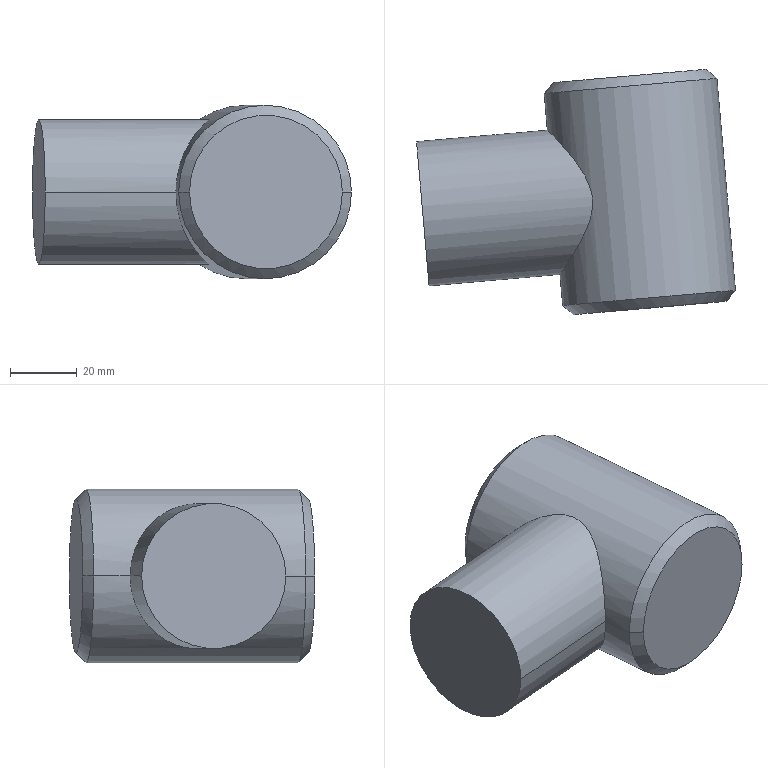Component | SolidWorks | RehabilitationChair-18-5-4 | 1 solid | 11 faces | box 95.66 x 73.56 x 52.03 mm | volume 209082 mm3 | cone 4 | cylinder 4 | plane 3 | commonest cylinder face diameters 43.427 x2 52.026 x2
STEP:
#1=CARTESIAN_POINT('',(7.385,20.16,15.393));
#2=VERTEX_POINT('',#1);
#3=CARTESIAN_POINT('',(9.191,20.318,15.393));
#4=VERTEX_POINT('',#3);
#5=CARTESIAN_POINT('',(8.288,20.239,15.393));
#6=DIRECTION('',(-0.08716,0.9962,0.00000002));
#7=DIRECTION('',(-0.9962,-0.08716,-0.00000001));
#8=AXIS2_PLACEMENT_3D('',#5,#6,#7);
#9=CIRCLE('',#8,0.906);
#10=EDGE_CURVE('',#2,#4,#9,.T.);
#11=ORIENTED_EDGE('',*,*,#10,.F.);
#12=CARTESIAN_POINT('',(7.278,20.032,15.393));
#13=VERTEX_POINT('',#12);
#14=CARTESIAN_POINT('',(7.385,20.16,15.393));
#15=DIRECTION('',(-0.6428,-0.766,-0.00000002));
#16=VECTOR('',#15,39.37);
#17=LINE('',#14,#16);
#18=EDGE_CURVE('',#2,#13,#17,.T.);
#19=ORIENTED_EDGE('',*,*,#18,.T.);
#20=CARTESIAN_POINT('',(9.319,20.21,15.393));
#21=VERTEX_POINT('',#20);
#22=CARTESIAN_POINT('',(8.298,20.121,15.393));
#23=DIRECTION('',(0.08716,-0.9962,-0.00000002));
#24=DIRECTION('',(-0.9962,-0.08716,-0.00000001));
#25=AXIS2_PLACEMENT_3D('',#22,#23,#24);
#26=CIRCLE('',#25,1.024);
#27=EDGE_CURVE('',#21,#13,#26,.T.);
#28=ORIENTED_EDGE('',*,*,#27,.F.);
#29=CARTESIAN_POINT('',(9.191,20.318,15.393));
#30=DIRECTION('',(0.766,-0.6428,-0.00000001));
#31=VECTOR('',#30,39.37);
#32=LINE('',#29,#31);
#33=EDGE_CURVE('',#4,#21,#32,.T.);
#34=ORIENTED_EDGE('',*,*,#33,.F.);
#35=EDGE_LOOP('',(#11,#19,#28,#34));
#36=FACE_OUTER_BOUND('',#35,.T.);
#37=CARTESIAN_POINT('',(8.288,20.239,15.393));
#38=DIRECTION('',(0.08716,-0.9962,-0.00000002));
#39=DIRECTION('',(0.9962,0.08716,0.00000001));
#40=AXIS2_PLACEMENT_3D('',#37,#38,#39);
#41=CONICAL_SURFACE('',#40,0.906,0.7854);
#42=ADVANCED_FACE('',(#36),#41,.T.);
#43=CARTESIAN_POINT('',(9.43,17.58,15.393));
#44=VERTEX_POINT('',#43);
#45=CARTESIAN_POINT('',(7.625,17.422,15.393));
#46=VERTEX_POINT('',#45);
#47=CARTESIAN_POINT('',(8.528,17.501,15.393));
#48=DIRECTION('',(0.08716,-0.9962,-0.00000002));
#49=DIRECTION('',(0.9962,0.08716,0.00000001));
#50=AXIS2_PLACEMENT_3D('',#47,#48,#49);
#51=CIRCLE('',#50,0.906);
#52=EDGE_CURVE('',#44,#46,#51,.T.);
#53=ORIENTED_EDGE('',*,*,#52,.F.);
#54=CARTESIAN_POINT('',(9.538,17.708,15.393));
#55=VERTEX_POINT('',#54);
#56=CARTESIAN_POINT('',(9.538,17.708,15.393));
#57=DIRECTION('',(0.6428,0.766,0.00000002));
#58=VECTOR('',#57,39.37);
#59=LINE('',#56,#58);
#60=EDGE_CURVE('',#44,#55,#59,.T.);
#61=ORIENTED_EDGE('',*,*,#60,.T.);
#62=CARTESIAN_POINT('',(7.497,17.529,15.393));
#63=VERTEX_POINT('',#62);
#64=CARTESIAN_POINT('',(8.517,17.618,15.393));
#65=DIRECTION('',(-0.08716,0.9962,0.00000002));
#66=DIRECTION('',(0.9962,0.08716,0.00000001));
#67=AXIS2_PLACEMENT_3D('',#64,#65,#66);
#68=CIRCLE('',#67,1.024);
#69=EDGE_CURVE('',#63,#55,#68,.T.);
#70=ORIENTED_EDGE('',*,*,#69,.F.);
#71=CARTESIAN_POINT('',(7.497,17.529,15.393));
#72=DIRECTION('',(-0.766,0.6428,0.00000001));
#73=VECTOR('',#72,39.37);
#74=LINE('',#71,#73);
#75=EDGE_CURVE('',#46,#63,#74,.T.);
#76=ORIENTED_EDGE('',*,*,#75,.F.);
#77=EDGE_LOOP('',(#53,#61,#70,#76));
#78=FACE_OUTER_BOUND('',#77,.T.);
#79=CARTESIAN_POINT('',(8.517,17.618,15.393));
#80=DIRECTION('',(-0.08716,0.9962,0.00000002));
#81=DIRECTION('',(-0.9962,-0.08716,-0.00000001));
#82=AXIS2_PLACEMENT_3D('',#79,#80,#81);
#83=CONICAL_SURFACE('',#82,1.024,0.7854);
#84=ADVANCED_FACE('',(#78),#83,.T.);
#85=CARTESIAN_POINT('',(5.771,19.464,15.393));
#86=VERTEX_POINT('',#85);
#87=CARTESIAN_POINT('',(5.92,17.761,15.393));
#88=VERTEX_POINT('',#87);
#89=CARTESIAN_POINT('',(5.846,18.613,15.393));
#90=DIRECTION('',(0.9962,0.08716,0.00000001));
#91=DIRECTION('',(0.08716,-0.9962,-0.00000002));
#92=AXIS2_PLACEMENT_3D('',#89,#90,#91);
#93=CIRCLE('',#92,0.8549);
#94=EDGE_CURVE('',#86,#88,#93,.T.);
#95=ORIENTED_EDGE('',*,*,#94,.T.);
#96=CARTESIAN_POINT('',(7.465,17.896,15.393));
#97=VERTEX_POINT('',#96);
#98=CARTESIAN_POINT('',(-5.673,16.747,15.393));
#99=DIRECTION('',(0.9962,0.08716,0.00000001));
#100=VECTOR('',#99,39.37);
#101=LINE('',#98,#100);
#102=EDGE_CURVE('',#88,#97,#101,.T.);
#103=ORIENTED_EDGE('',*,*,#102,.T.);
#104=CARTESIAN_POINT('',(7.316,19.6,15.393));
#105=VERTEX_POINT('',#104);
#106=CARTESIAN_POINT('',(7.316,19.6,15.393));
#107=CARTESIAN_POINT('',(7.316,19.6,15.454));
#108=CARTESIAN_POINT('',(7.322,19.594,15.513));
#109=CARTESIAN_POINT('',(7.336,19.58,15.585));
#110=CARTESIAN_POINT('',(7.339,19.576,15.599));
#111=CARTESIAN_POINT('',(7.346,19.569,15.627));
#112=CARTESIAN_POINT('',(7.349,19.566,15.641));
#113=CARTESIAN_POINT('',(7.362,19.553,15.683));
#114=CARTESIAN_POINT('',(7.371,19.544,15.71));
#115=CARTESIAN_POINT('',(7.391,19.523,15.762));
#116=CARTESIAN_POINT('',(7.402,19.511,15.787));
#117=CARTESIAN_POINT('',(7.427,19.486,15.836));
#118=CARTESIAN_POINT('',(7.44,19.472,15.859));
#119=CARTESIAN_POINT('',(7.48,19.428,15.927));
#120=CARTESIAN_POINT('',(7.509,19.396,15.967));
#121=CARTESIAN_POINT('',(7.555,19.343,16.023));
#122=CARTESIAN_POINT('',(7.571,19.325,16.04));
#123=CARTESIAN_POINT('',(7.603,19.286,16.074));
#124=CARTESIAN_POINT('',(7.619,19.267,16.089));
#125=CARTESIAN_POINT('',(7.667,19.205,16.133));
#126=CARTESIAN_POINT('',(7.698,19.161,16.158));
#127=CARTESIAN_POINT('',(7.735,19.102,16.185));
#128=CARTESIAN_POINT('',(7.743,19.09,16.19));
#129=CARTESIAN_POINT('',(7.757,19.065,16.199));
#130=CARTESIAN_POINT('',(7.764,19.053,16.204));
#131=CARTESIAN_POINT('',(7.784,19.014,16.217));
#132=CARTESIAN_POINT('',(7.796,18.988,16.224));
#133=CARTESIAN_POINT('',(7.812,18.947,16.233));
#134=CARTESIAN_POINT('',(7.817,18.933,16.235));
#135=CARTESIAN_POINT('',(7.826,18.905,16.24));
#136=CARTESIAN_POINT('',(7.831,18.89,16.242));
#137=CARTESIAN_POINT('',(7.841,18.847,16.247));
#138=CARTESIAN_POINT('',(7.846,18.817,16.248));
#139=CARTESIAN_POINT('',(7.851,18.758,16.248));
#140=CARTESIAN_POINT('',(7.852,18.728,16.246));
#141=CARTESIAN_POINT('',(7.848,18.668,16.24));
#142=CARTESIAN_POINT('',(7.843,18.639,16.236));
#143=CARTESIAN_POINT('',(7.832,18.581,16.224));
#144=CARTESIAN_POINT('',(7.824,18.553,16.216));
#145=CARTESIAN_POINT('',(7.811,18.512,16.204));
#146=CARTESIAN_POINT('',(7.806,18.498,16.199));
#147=CARTESIAN_POINT('',(7.796,18.472,16.19));
#148=CARTESIAN_POINT('',(7.791,18.458,16.185));
#149=CARTESIAN_POINT('',(7.765,18.394,16.158));
#150=CARTESIAN_POINT('',(7.742,18.345,16.133));
#151=CARTESIAN_POINT('',(7.705,18.276,16.089));
#152=CARTESIAN_POINT('',(7.693,18.254,16.073));
#153=CARTESIAN_POINT('',(7.668,18.21,16.04));
#154=CARTESIAN_POINT('',(7.656,18.189,16.022));
#155=CARTESIAN_POINT('',(7.62,18.13,15.967));
#156=CARTESIAN_POINT('',(7.596,18.093,15.926));
#157=CARTESIAN_POINT('',(7.564,18.043,15.859));
#158=CARTESIAN_POINT('',(7.554,18.027,15.835));
#159=CARTESIAN_POINT('',(7.535,17.998,15.786));
#160=CARTESIAN_POINT('',(7.526,17.985,15.761));
#161=CARTESIAN_POINT('',(7.509,17.961,15.709));
#162=CARTESIAN_POINT('',(7.502,17.95,15.683));
#163=CARTESIAN_POINT('',(7.489,17.931,15.627));
#164=CARTESIAN_POINT('',(7.483,17.923,15.599));
#165=CARTESIAN_POINT('',(7.47,17.903,15.512));
#166=CARTESIAN_POINT('',(7.465,17.896,15.453));
#167=CARTESIAN_POINT('',(7.465,17.896,15.393));
#168=B_SPLINE_CURVE_WITH_KNOTS('',3,(#106,#107,#108,#109,#110,#111,#112,#113,#114,#115,#116,#117,#118,#119,#120,#121,#122,#123,#124,#125,#126,#127,#128,#129,#130,#131,#132,#133,#134,#135,#136,#137,#138,#139,#140,#141,#142,#143,#144,#145,#146,#147,#148,#149,#150,#151,#152,#153,#154,#155,#156,#157,#158,#159,#160,#161,#162,#163,#164,#165,#166,#167),.UNSPECIFIED.,.F.,.F.,(4,2,2,2,2,2,2,2,2,2,2,2,2,2,2,2,2,2,2,2,2,2,2,2,2,2,2,2,2,2,4),(0.,0.004533,0.005667,0.0068,0.009067,0.01133,0.0136,0.01813,0.0204,0.02267,0.0272,0.02833,0.02947,0.03173,0.03287,0.034,0.03627,0.03853,0.0408,0.04307,0.0442,0.04533,0.04987,0.05213,0.0544,0.05893,0.0612,0.06347,0.06573,0.068,0.07253),.UNSPECIFIED.);
#169=EDGE_CURVE('',#105,#97,#168,.T.);
#170=ORIENTED_EDGE('',*,*,#169,.F.);
#171=CARTESIAN_POINT('',(-5.822,18.45,15.393));
#172=DIRECTION('',(0.9962,0.08716,0.00000001));
#173=VECTOR('',#172,39.37);
#174=LINE('',#171,#173);
#175=EDGE_CURVE('',#86,#105,#174,.T.);
#176=ORIENTED_EDGE('',*,*,#175,.F.);
#177=EDGE_LOOP('',(#95,#103,#170,#176));
#178=FACE_OUTER_BOUND('',#177,.T.);
#179=CARTESIAN_POINT('',(-5.748,17.598,15.393));
#180=DIRECTION('',(0.9962,0.08716,0.00000001));
#181=DIRECTION('',(-0.08716,0.9962,0.00000002));
#182=AXIS2_PLACEMENT_3D('',#179,#180,#181);
#183=CYLINDRICAL_SURFACE('',#182,0.8549);
#184=ADVANCED_FACE('',(#178),#183,.T.);
#185=ORIENTED_EDGE('',*,*,#69,.T.);
#186=CARTESIAN_POINT('',(9.308,20.328,15.393));
#187=DIRECTION('',(-0.08716,0.9962,0.00000002));
#188=VECTOR('',#187,39.37);
#189=LINE('',#186,#188);
#190=EDGE_CURVE('',#55,#21,#189,.T.);
#191=ORIENTED_EDGE('',*,*,#190,.T.);
#192=ORIENTED_EDGE('',*,*,#27,.T.);
#193=CARTESIAN_POINT('',(7.268,20.15,15.393));
#194=DIRECTION('',(-0.08716,0.9962,0.00000002));
#195=VECTOR('',#194,39.37);
#196=LINE('',#193,#195);
#197=EDGE_CURVE('',#105,#13,#196,.T.);
#198=ORIENTED_EDGE('',*,*,#197,.F.);
#199=ORIENTED_EDGE('',*,*,#169,.T.);
#200=CARTESIAN_POINT('',(7.268,20.15,15.393));
#201=DIRECTION('',(-0.08716,0.9962,0.00000002));
#202=VECTOR('',#201,39.37);
#203=LINE('',#200,#202);
#204=EDGE_CURVE('',#63,#97,#203,.T.);
#205=ORIENTED_EDGE('',*,*,#204,.F.);
#206=EDGE_LOOP('',(#185,#191,#192,#198,#199,#205));
#207=FACE_OUTER_BOUND('',#206,.T.);
#208=CARTESIAN_POINT('',(8.288,20.239,15.393));
#209=DIRECTION('',(-0.08716,0.9962,0.00000002));
#210=DIRECTION('',(-0.9962,-0.08716,-0.00000001));
#211=AXIS2_PLACEMENT_3D('',#208,#209,#210);
#212=CYLINDRICAL_SURFACE('',#211,1.024);
#213=ADVANCED_FACE('',(#207),#212,.T.);
#214=CARTESIAN_POINT('',(8.288,20.239,15.393));
#215=DIRECTION('',(-0.08716,0.9962,0.00000002));
#216=DIRECTION('',(-0.9962,-0.08716,-0.00000001));
#217=AXIS2_PLACEMENT_3D('',#214,#215,#216);
#218=CIRCLE('',#217,0.906);
#219=EDGE_CURVE('',#4,#2,#218,.T.);
#220=ORIENTED_EDGE('',*,*,#219,.T.);
#221=ORIENTED_EDGE('',*,*,#10,.T.);
#222=EDGE_LOOP('',(#220,#221));
#223=FACE_OUTER_BOUND('',#222,.T.);
#224=CARTESIAN_POINT('',(8.288,20.239,15.393));
#225=DIRECTION('',(-0.08716,0.9962,0.00000002));
#226=DIRECTION('',(-0.9962,-0.08716,-0.00000001));
#227=AXIS2_PLACEMENT_3D('',#224,#225,#226);
#228=PLANE('',#227);
#229=ADVANCED_FACE('',(#223),#228,.T.);
#230=CARTESIAN_POINT('',(8.528,17.501,15.393));
#231=DIRECTION('',(0.08716,-0.9962,-0.00000002));
#232=DIRECTION('',(0.9962,0.08716,0.00000001));
#233=AXIS2_PLACEMENT_3D('',#230,#231,#232);
#234=CIRCLE('',#233,0.906);
#235=EDGE_CURVE('',#46,#44,#234,.T.);
#236=ORIENTED_EDGE('',*,*,#235,.T.);
#237=ORIENTED_EDGE('',*,*,#52,.T.);
#238=EDGE_LOOP('',(#236,#237));
#239=FACE_OUTER_BOUND('',#238,.T.);
#240=CARTESIAN_POINT('',(8.528,17.501,15.393));
#241=DIRECTION('',(0.08716,-0.9962,-0.00000002));
#242=DIRECTION('',(0.9962,0.08716,0.00000001));
#243=AXIS2_PLACEMENT_3D('',#240,#241,#242);
#244=PLANE('',#243);
#245=ADVANCED_FACE('',(#239),#244,.T.);
#246=ORIENTED_EDGE('',*,*,#190,.F.);
#247=CARTESIAN_POINT('',(8.517,17.618,15.393));
#248=DIRECTION('',(-0.08716,0.9962,0.00000002));
#249=DIRECTION('',(0.9962,0.08716,0.00000001));
#250=AXIS2_PLACEMENT_3D('',#247,#248,#249);
#251=CIRCLE('',#250,1.024);
#252=EDGE_CURVE('',#55,#63,#251,.T.);
#253=ORIENTED_EDGE('',*,*,#252,.T.);
#254=ORIENTED_EDGE('',*,*,#204,.T.);
#255=CARTESIAN_POINT('',(7.465,17.896,15.393));
#256=CARTESIAN_POINT('',(7.465,17.896,15.378));
#257=CARTESIAN_POINT('',(7.465,17.897,15.363));
#258=CARTESIAN_POINT('',(7.466,17.898,15.333));
#259=CARTESIAN_POINT('',(7.467,17.9,15.318));
#260=CARTESIAN_POINT('',(7.471,17.905,15.274));
#261=CARTESIAN_POINT('',(7.474,17.91,15.244));
#262=CARTESIAN_POINT('',(7.481,17.919,15.201));
#263=CARTESIAN_POINT('',(7.484,17.923,15.187));
#264=CARTESIAN_POINT('',(7.489,17.931,15.159));
#265=CARTESIAN_POINT('',(7.492,17.936,15.145));
#266=CARTESIAN_POINT('',(7.502,17.95,15.103));
#267=CARTESIAN_POINT('',(7.509,17.961,15.076));
#268=CARTESIAN_POINT('',(7.526,17.985,15.024));
#269=CARTESIAN_POINT('',(7.535,17.999,14.999));
#270=CARTESIAN_POINT('',(7.554,18.028,14.95));
#271=CARTESIAN_POINT('',(7.565,18.044,14.927));
#272=CARTESIAN_POINT('',(7.597,18.094,14.859));
#273=CARTESIAN_POINT('',(7.62,18.13,14.819));
#274=CARTESIAN_POINT('',(7.656,18.19,14.763));
#275=CARTESIAN_POINT('',(7.669,18.211,14.746));
#276=CARTESIAN_POINT('',(7.693,18.255,14.713));
#277=CARTESIAN_POINT('',(7.706,18.277,14.697));
#278=CARTESIAN_POINT('',(7.742,18.346,14.653));
#279=CARTESIAN_POINT('',(7.765,18.394,14.628));
#280=CARTESIAN_POINT('',(7.797,18.472,14.596));
#281=CARTESIAN_POINT('',(7.807,18.499,14.587));
#282=CARTESIAN_POINT('',(7.824,18.554,14.57));
#283=CARTESIAN_POINT('',(7.832,18.582,14.562));
#284=CARTESIAN_POINT('',(7.843,18.639,14.551));
#285=CARTESIAN_POINT('',(7.848,18.669,14.546));
#286=CARTESIAN_POINT('',(7.852,18.729,14.54));
#287=CARTESIAN_POINT('',(7.851,18.759,14.538));
#288=CARTESIAN_POINT('',(7.846,18.818,14.538));
#289=CARTESIAN_POINT('',(7.841,18.847,14.54));
#290=CARTESIAN_POINT('',(7.827,18.906,14.546));
#291=CARTESIAN_POINT('',(7.818,18.934,14.551));
#292=CARTESIAN_POINT('',(7.796,18.988,14.563));
#293=CARTESIAN_POINT('',(7.784,19.015,14.57));
#294=CARTESIAN_POINT('',(7.764,19.053,14.582));
#295=CARTESIAN_POINT('',(7.757,19.066,14.587));
#296=CARTESIAN_POINT('',(7.742,19.09,14.596));
#297=CARTESIAN_POINT('',(7.735,19.102,14.602));
#298=CARTESIAN_POINT('',(7.698,19.161,14.628));
#299=CARTESIAN_POINT('',(7.667,19.205,14.653));
#300=CARTESIAN_POINT('',(7.619,19.267,14.697));
#301=CARTESIAN_POINT('',(7.603,19.287,14.713));
#302=CARTESIAN_POINT('',(7.571,19.325,14.746));
#303=CARTESIAN_POINT('',(7.555,19.344,14.764));
#304=CARTESIAN_POINT('',(7.509,19.396,14.819));
#305=CARTESIAN_POINT('',(7.48,19.429,14.86));
#306=CARTESIAN_POINT('',(7.446,19.465,14.916));
#307=CARTESIAN_POINT('',(7.44,19.472,14.927));
#308=CARTESIAN_POINT('',(7.427,19.485,14.951));
#309=CARTESIAN_POINT('',(7.421,19.492,14.963));
#310=CARTESIAN_POINT('',(7.402,19.511,14.999));
#311=CARTESIAN_POINT('',(7.391,19.523,15.024));
#312=CARTESIAN_POINT('',(7.371,19.544,15.076));
#313=CARTESIAN_POINT('',(7.362,19.553,15.103));
#314=CARTESIAN_POINT('',(7.346,19.57,15.158));
#315=CARTESIAN_POINT('',(7.339,19.577,15.187));
#316=CARTESIAN_POINT('',(7.322,19.594,15.274));
#317=CARTESIAN_POINT('',(7.316,19.6,15.333));
#318=CARTESIAN_POINT('',(7.316,19.6,15.393));
#319=B_SPLINE_CURVE_WITH_KNOTS('',3,(#255,#256,#257,#258,#259,#260,#261,#262,#263,#264,#265,#266,#267,#268,#269,#270,#271,#272,#273,#274,#275,#276,#277,#278,#279,#280,#281,#282,#283,#284,#285,#286,#287,#288,#289,#290,#291,#292,#293,#294,#295,#296,#297,#298,#299,#300,#301,#302,#303,#304,#305,#306,#307,#308,#309,#310,#311,#312,#313,#314,#315,#316,#317,#318),.UNSPECIFIED.,.F.,.F.,(4,2,2,2,2,2,2,2,2,2,2,2,2,2,2,2,2,2,2,2,2,2,2,2,2,2,2,2,2,2,2,4),(0.07253,0.07367,0.0748,0.07706,0.07819,0.07933,0.08159,0.08385,0.08612,0.09065,0.09291,0.09517,0.0997,0.102,0.1042,0.1065,0.1088,0.111,0.1133,0.1155,0.1167,0.1178,0.1223,0.1246,0.1269,0.1314,0.1325,0.1337,0.1359,0.1382,0.1405,0.145),.UNSPECIFIED.);
#320=EDGE_CURVE('',#97,#105,#319,.T.);
#321=ORIENTED_EDGE('',*,*,#320,.T.);
#322=ORIENTED_EDGE('',*,*,#197,.T.);
#323=CARTESIAN_POINT('',(8.298,20.121,15.393));
#324=DIRECTION('',(0.08716,-0.9962,-0.00000002));
#325=DIRECTION('',(-0.9962,-0.08716,-0.00000001));
#326=AXIS2_PLACEMENT_3D('',#323,#324,#325);
#327=CIRCLE('',#326,1.024);
#328=EDGE_CURVE('',#13,#21,#327,.T.);
#329=ORIENTED_EDGE('',*,*,#328,.T.);
#330=EDGE_LOOP('',(#246,#253,#254,#321,#322,#329));
#331=FACE_OUTER_BOUND('',#330,.T.);
#332=CARTESIAN_POINT('',(8.288,20.239,15.393));
#333=DIRECTION('',(-0.08716,0.9962,0.00000002));
#334=DIRECTION('',(-0.9962,-0.08716,-0.00000001));
#335=AXIS2_PLACEMENT_3D('',#332,#333,#334);
#336=CYLINDRICAL_SURFACE('',#335,1.024);
#337=ADVANCED_FACE('',(#331),#336,.T.);
#338=ORIENTED_EDGE('',*,*,#102,.F.);
#339=CARTESIAN_POINT('',(5.846,18.613,15.393));
#340=DIRECTION('',(0.9962,0.08716,0.00000001));
#341=DIRECTION('',(0.08716,-0.9962,-0.00000002));
#342=AXIS2_PLACEMENT_3D('',#339,#340,#341);
#343=CIRCLE('',#342,0.8549);
#344=EDGE_CURVE('',#88,#86,#343,.T.);
#345=ORIENTED_EDGE('',*,*,#344,.T.);
#346=ORIENTED_EDGE('',*,*,#175,.T.);
#347=ORIENTED_EDGE('',*,*,#320,.F.);
#348=EDGE_LOOP('',(#338,#345,#346,#347));
#349=FACE_OUTER_BOUND('',#348,.T.);
#350=CARTESIAN_POINT('',(-5.748,17.598,15.393));
#351=DIRECTION('',(0.9962,0.08716,0.00000001));
#352=DIRECTION('',(-0.08716,0.9962,0.00000002));
#353=AXIS2_PLACEMENT_3D('',#350,#351,#352);
#354=CYLINDRICAL_SURFACE('',#353,0.8549);
#355=ADVANCED_FACE('',(#349),#354,.T.);
#356=ORIENTED_EDGE('',*,*,#94,.F.);
#357=ORIENTED_EDGE('',*,*,#344,.F.);
#358=EDGE_LOOP('',(#356,#357));
#359=FACE_OUTER_BOUND('',#358,.T.);
#360=CARTESIAN_POINT('',(8.231,-8.646,13.025));
#361=DIRECTION('',(-0.9962,-0.08716,-0.00000001));
#362=DIRECTION('',(0.08716,-0.9962,-0.00000002));
#363=AXIS2_PLACEMENT_3D('',#360,#361,#362);
#364=PLANE('',#363);
#365=ADVANCED_FACE('',(#359),#364,.T.);
#366=ORIENTED_EDGE('',*,*,#60,.F.);
#367=ORIENTED_EDGE('',*,*,#235,.F.);
#368=ORIENTED_EDGE('',*,*,#75,.T.);
#369=ORIENTED_EDGE('',*,*,#252,.F.);
#370=EDGE_LOOP('',(#366,#367,#368,#369));
#371=FACE_OUTER_BOUND('',#370,.T.);
#372=CARTESIAN_POINT('',(8.517,17.618,15.393));
#373=DIRECTION('',(-0.08716,0.9962,0.00000002));
#374=DIRECTION('',(-0.9962,-0.08716,-0.00000001));
#375=AXIS2_PLACEMENT_3D('',#372,#373,#374);
#376=CONICAL_SURFACE('',#375,1.024,0.7854);
#377=ADVANCED_FACE('',(#371),#376,.T.);
#378=ORIENTED_EDGE('',*,*,#18,.F.);
#379=ORIENTED_EDGE('',*,*,#219,.F.);
#380=ORIENTED_EDGE('',*,*,#33,.T.);
#381=ORIENTED_EDGE('',*,*,#328,.F.);
#382=EDGE_LOOP('',(#378,#379,#380,#381));
#383=FACE_OUTER_BOUND('',#382,.T.);
#384=CARTESIAN_POINT('',(8.288,20.239,15.393));
#385=DIRECTION('',(0.08716,-0.9962,-0.00000002));
#386=DIRECTION('',(0.9962,0.08716,0.00000001));
#387=AXIS2_PLACEMENT_3D('',#384,#385,#386);
#388=CONICAL_SURFACE('',#387,0.906,0.7854);
#389=ADVANCED_FACE('',(#383),#388,.T.);
#390=CLOSED_SHELL('',(#42,#84,#184,#213,#229,#245,#337,#355,#365,#377,#389));
#391=MANIFOLD_SOLID_BREP('',#390);
#392=CARTESIAN_POINT('',(0.,0.,0.));
#393=DIRECTION('',(0.,0.,1.));
#394=DIRECTION('',(1.,0.,0.));
#395=AXIS2_PLACEMENT_3D('',#392,#393,#394);
#396=(LENGTH_UNIT()NAMED_UNIT(*)SI_UNIT($,.METRE.));
#397=LENGTH_MEASURE_WITH_UNIT(LENGTH_MEASURE(0.0254),#396);
#398=DIMENSIONAL_EXPONENTS(1.,0.,0.,0.,0.,0.,0.);
#399=(CONVERSION_BASED_UNIT('',#397)LENGTH_UNIT()NAMED_UNIT(#398));
#400=UNCERTAINTY_MEASURE_WITH_UNIT(LENGTH_MEASURE(0.00001),#399,'','');
#401=(NAMED_UNIT(*)PLANE_ANGLE_UNIT()SI_UNIT($,.RADIAN.));
#402=(NAMED_UNIT(*)SI_UNIT($,.STERADIAN.)SOLID_ANGLE_UNIT());
#403=(GEOMETRIC_REPRESENTATION_CONTEXT(3)GLOBAL_UNCERTAINTY_ASSIGNED_CONTEXT((#400))GLOBAL_UNIT_ASSIGNED_CONTEXT((#399,#401,#402))REPRESENTATION_CONTEXT('',''));
#404=ADVANCED_BREP_SHAPE_REPRESENTATION('',(#391,#395),#403);
#405=COLOUR_RGB('',0.7922,0.8196,0.9333);
#406=FILL_AREA_STYLE_COLOUR('',#405);
#407=FILL_AREA_STYLE('',(#406));
#408=SURFACE_STYLE_FILL_AREA(#407);
#409=SURFACE_SIDE_STYLE('',(#408));
#410=SURFACE_STYLE_USAGE(.BOTH.,#409);
#411=PRESENTATION_STYLE_ASSIGNMENT((#410));
#412=STYLED_ITEM('',(#411),#391);
#413=(LENGTH_UNIT()NAMED_UNIT(*)SI_UNIT($,.METRE.));
#414=LENGTH_MEASURE_WITH_UNIT(LENGTH_MEASURE(0.0254),#413);
#415=DIMENSIONAL_EXPONENTS(1.,0.,0.,0.,0.,0.,0.);
#416=(CONVERSION_BASED_UNIT('',#414)LENGTH_UNIT()NAMED_UNIT(#415));
#417=UNCERTAINTY_MEASURE_WITH_UNIT(LENGTH_MEASURE(0.00001),#416,'','');
#418=(NAMED_UNIT(*)PLANE_ANGLE_UNIT()SI_UNIT($,.RADIAN.));
#419=(NAMED_UNIT(*)SI_UNIT($,.STERADIAN.)SOLID_ANGLE_UNIT());
#420=(GEOMETRIC_REPRESENTATION_CONTEXT(3)GLOBAL_UNCERTAINTY_ASSIGNED_CONTEXT((#417))GLOBAL_UNIT_ASSIGNED_CONTEXT((#416,#418,#419))REPRESENTATION_CONTEXT('',''));
#421=MECHANICAL_DESIGN_GEOMETRIC_PRESENTATION_REPRESENTATION('',(#412),#420);
#422=PRESENTATION_LAYER_ASSIGNMENT('','',(#412));